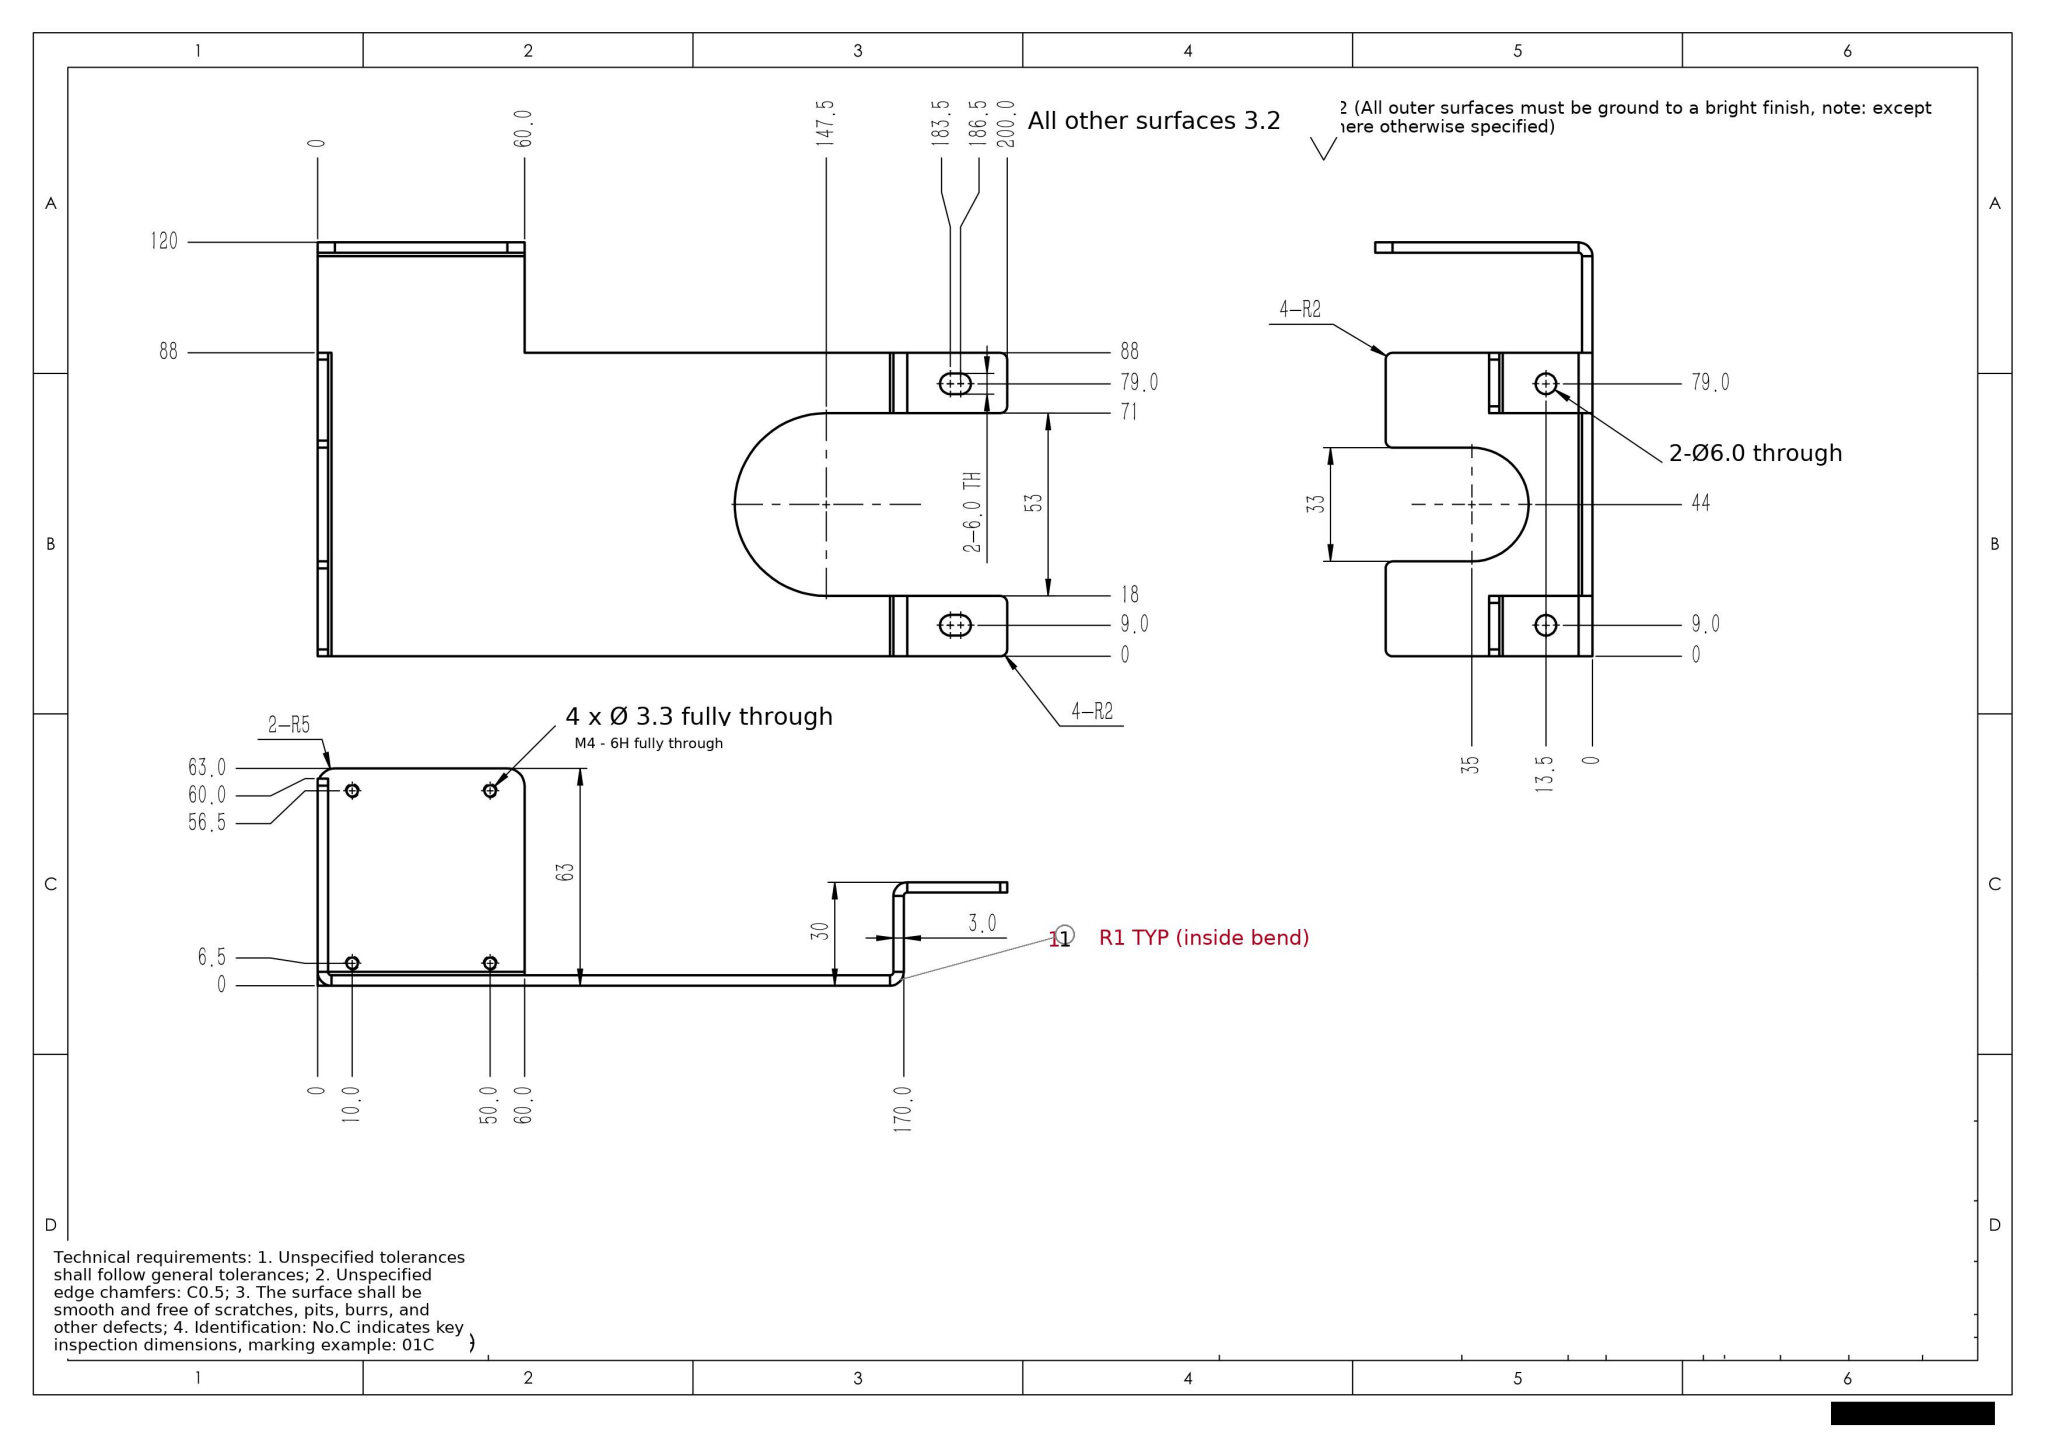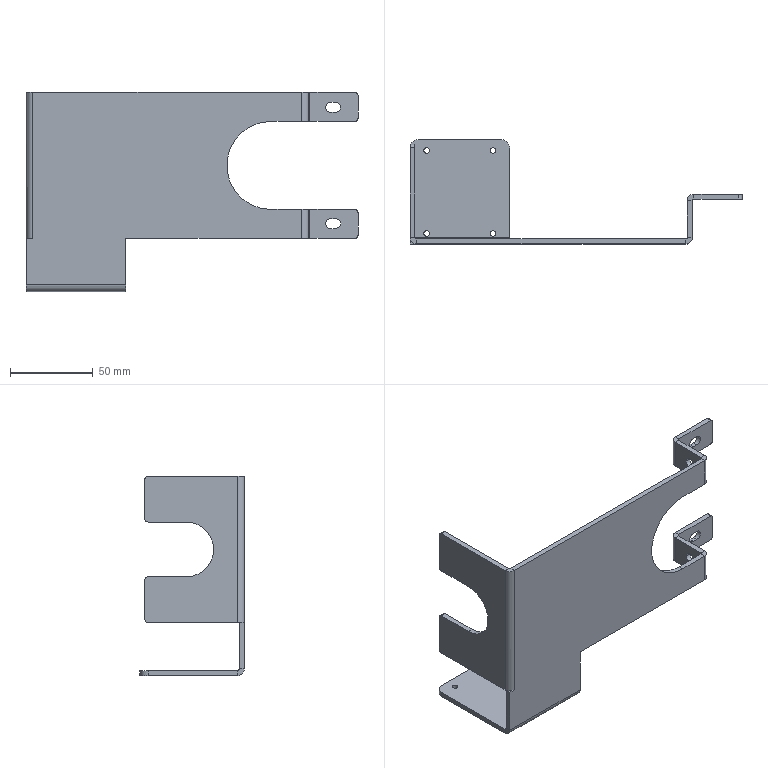Part | SolidWorks | mm | 1 solid | 99 faces | box 200 x 63 x 120 mm | volume 70524 mm3 | plane 56 | cylinder 43 | commonest cylinder face diameters 6 x10 3.3 x8 4 x8 8 x6 2 x6 33 x2 10 x2 53 x1